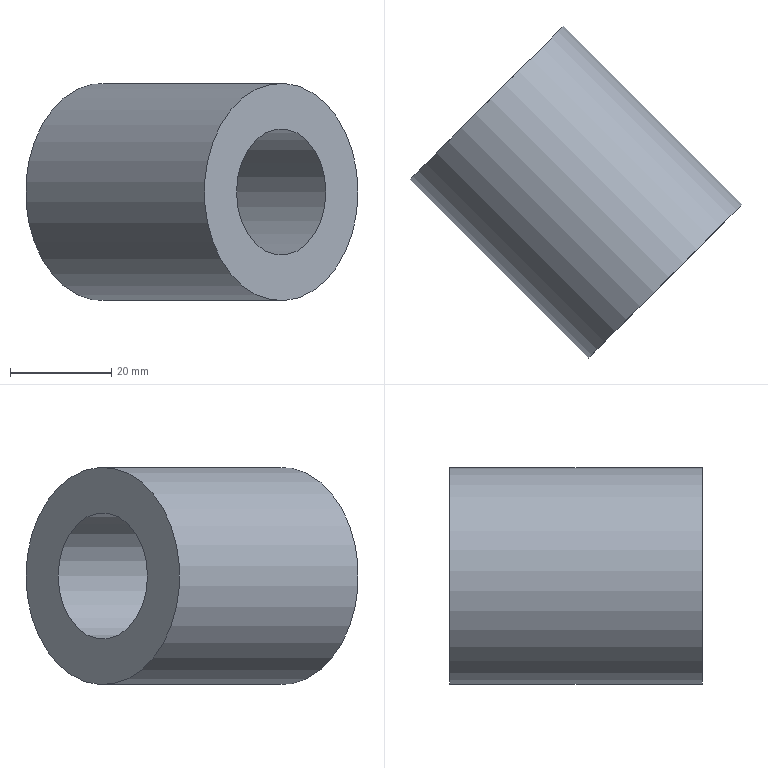Component | NX | INCL_SUPP_FRAME_CONN_COL_2 | 1 solid | 4 faces | box 65.76 x 65.76 x 43 mm | volume 48066 mm3 | cylinder 2 | plane 2 | commonest cylinder face diameters 43 x1 25 x1
STEP:
#1=CARTESIAN_POINT('',(0.,0.,0.));
#2=DIRECTION('',(0.,0.,1.));
#3=DIRECTION('',(1.,0.,0.));
#4=AXIS2_PLACEMENT_3D('',#1,#2,#3);
#5=CARTESIAN_POINT('',(-786.016,863.173,-601.5));
#6=VERTEX_POINT('',#5);
#7=CARTESIAN_POINT('',(-801.219,847.97,-601.5));
#8=DIRECTION('',(0.7071,-0.7071,0.));
#9=DIRECTION('',(0.7071,0.7071,0.));
#10=AXIS2_PLACEMENT_3D('',#7,#8,#9);
#11=CIRCLE('',#10,21.5);
#12=CARTESIAN_POINT('',(-801.219,847.97,-601.5));
#13=DIRECTION('',(0.7071,-0.7071,0.));
#14=DIRECTION('',(-0.7071,-0.7071,0.));
#15=AXIS2_PLACEMENT_3D('',#12,#13,#14);
#16=CYLINDRICAL_SURFACE('',#15,21.5);
#17=CARTESIAN_POINT('',(3.142,0.));
#18=DIRECTION('',(1.,0.));
#19=VECTOR('',#18,1.);
#20=LINE('',#17,#19);
#21=(GEOMETRIC_REPRESENTATION_CONTEXT(2)PARAMETRIC_REPRESENTATION_CONTEXT()REPRESENTATION_CONTEXT('',''));
#22=DEFINITIONAL_REPRESENTATION('',(#20),#21);
#23=PCURVE('',#16,#22);
#24=CARTESIAN_POINT('',(-801.219,847.97,-601.5));
#25=DIRECTION('',(0.7071,-0.7071,0.));
#26=DIRECTION('',(-0.7071,-0.7071,0.));
#27=AXIS2_PLACEMENT_3D('',#24,#25,#26);
#28=PLANE('',#27);
#29=CARTESIAN_POINT('',(0.,0.));
#30=DIRECTION('',(-1.,0.));
#31=AXIS2_PLACEMENT_2D('',#29,#30);
#32=CIRCLE('',#31,21.5);
#33=(GEOMETRIC_REPRESENTATION_CONTEXT(2)PARAMETRIC_REPRESENTATION_CONTEXT()REPRESENTATION_CONTEXT('',''));
#34=DEFINITIONAL_REPRESENTATION('',(#32),#33);
#35=PCURVE('',#28,#34);
#36=SURFACE_CURVE('',#11,(#23,#35),.PCURVE_S1.);
#37=EDGE_CURVE('',#6,#6,#36,.T.);
#38=ORIENTED_EDGE('',*,*,#37,.T.);
#39=CARTESIAN_POINT('',(-750.661,827.817,-601.5));
#40=VERTEX_POINT('',#39);
#41=CARTESIAN_POINT('',(-786.016,863.173,-601.5));
#42=CARTESIAN_POINT('',(-750.661,827.817,-601.5));
#43=B_SPLINE_CURVE_WITH_KNOTS('',1,(#41,#42),.UNSPECIFIED.,.F.,.F.,(2,2),(0.,50.),.PIECEWISE_BEZIER_KNOTS.);
#44=CARTESIAN_POINT('',(9.425,0.));
#45=DIRECTION('',(0.,1.));
#46=VECTOR('',#45,1.);
#47=LINE('',#44,#46);
#48=(GEOMETRIC_REPRESENTATION_CONTEXT(2)PARAMETRIC_REPRESENTATION_CONTEXT()REPRESENTATION_CONTEXT('',''));
#49=DEFINITIONAL_REPRESENTATION('',(#47),#48);
#50=PCURVE('',#16,#49);
#51=CARTESIAN_POINT('',(3.142,0.));
#52=DIRECTION('',(0.,1.));
#53=VECTOR('',#52,1.);
#54=LINE('',#51,#53);
#55=(GEOMETRIC_REPRESENTATION_CONTEXT(2)PARAMETRIC_REPRESENTATION_CONTEXT()REPRESENTATION_CONTEXT('',''));
#56=DEFINITIONAL_REPRESENTATION('',(#54),#55);
#57=PCURVE('',#16,#56);
#58=SEAM_CURVE('',#43,(#50,#57),.PCURVE_S1.);
#59=EDGE_CURVE('',#6,#40,#58,.T.);
#60=ORIENTED_EDGE('',*,*,#59,.T.);
#61=CARTESIAN_POINT('',(-765.864,812.615,-601.5));
#62=DIRECTION('',(0.7071,-0.7071,0.));
#63=DIRECTION('',(0.7071,0.7071,0.));
#64=AXIS2_PLACEMENT_3D('',#61,#62,#63);
#65=CIRCLE('',#64,21.5);
#66=CARTESIAN_POINT('',(3.142,50.));
#67=DIRECTION('',(1.,0.));
#68=VECTOR('',#67,1.);
#69=LINE('',#66,#68);
#70=(GEOMETRIC_REPRESENTATION_CONTEXT(2)PARAMETRIC_REPRESENTATION_CONTEXT()REPRESENTATION_CONTEXT('',''));
#71=DEFINITIONAL_REPRESENTATION('',(#69),#70);
#72=PCURVE('',#16,#71);
#73=CARTESIAN_POINT('',(-765.864,812.615,-601.5));
#74=DIRECTION('',(0.7071,-0.7071,0.));
#75=DIRECTION('',(-0.7071,-0.7071,0.));
#76=AXIS2_PLACEMENT_3D('',#73,#74,#75);
#77=PLANE('',#76);
#78=CARTESIAN_POINT('',(0.,0.));
#79=DIRECTION('',(-1.,0.));
#80=AXIS2_PLACEMENT_2D('',#78,#79);
#81=CIRCLE('',#80,21.5);
#82=(GEOMETRIC_REPRESENTATION_CONTEXT(2)PARAMETRIC_REPRESENTATION_CONTEXT()REPRESENTATION_CONTEXT('',''));
#83=DEFINITIONAL_REPRESENTATION('',(#81),#82);
#84=PCURVE('',#77,#83);
#85=SURFACE_CURVE('',#65,(#72,#84),.PCURVE_S1.);
#86=EDGE_CURVE('',#40,#40,#85,.T.);
#87=ORIENTED_EDGE('',*,*,#86,.F.);
#88=ORIENTED_EDGE('',*,*,#59,.F.);
#89=EDGE_LOOP('',(#38,#60,#87,#88));
#90=FACE_BOUND('',#89,.T.);
#91=ADVANCED_FACE('',(#90),#16,.T.);
#92=CARTESIAN_POINT('',(-792.38,856.809,-601.5));
#93=VERTEX_POINT('',#92);
#94=CARTESIAN_POINT('',(-801.219,847.97,-601.5));
#95=DIRECTION('',(0.7071,-0.7071,0.));
#96=DIRECTION('',(0.7071,0.7071,0.));
#97=AXIS2_PLACEMENT_3D('',#94,#95,#96);
#98=CIRCLE('',#97,12.5);
#99=CARTESIAN_POINT('',(-801.219,847.97,-601.5));
#100=DIRECTION('',(0.7071,-0.7071,0.));
#101=DIRECTION('',(-0.7071,-0.7071,0.));
#102=AXIS2_PLACEMENT_3D('',#99,#100,#101);
#103=CYLINDRICAL_SURFACE('',#102,12.5);
#104=CARTESIAN_POINT('',(3.142,0.));
#105=DIRECTION('',(1.,0.));
#106=VECTOR('',#105,1.);
#107=LINE('',#104,#106);
#108=(GEOMETRIC_REPRESENTATION_CONTEXT(2)PARAMETRIC_REPRESENTATION_CONTEXT()REPRESENTATION_CONTEXT('',''));
#109=DEFINITIONAL_REPRESENTATION('',(#107),#108);
#110=PCURVE('',#103,#109);
#111=CARTESIAN_POINT('',(0.,0.));
#112=DIRECTION('',(-1.,0.));
#113=AXIS2_PLACEMENT_2D('',#111,#112);
#114=CIRCLE('',#113,12.5);
#115=(GEOMETRIC_REPRESENTATION_CONTEXT(2)PARAMETRIC_REPRESENTATION_CONTEXT()REPRESENTATION_CONTEXT('',''));
#116=DEFINITIONAL_REPRESENTATION('',(#114),#115);
#117=PCURVE('',#28,#116);
#118=SURFACE_CURVE('',#98,(#110,#117),.PCURVE_S1.);
#119=EDGE_CURVE('',#93,#93,#118,.T.);
#120=ORIENTED_EDGE('',*,*,#119,.T.);
#121=CARTESIAN_POINT('',(-757.025,821.453,-601.5));
#122=VERTEX_POINT('',#121);
#123=CARTESIAN_POINT('',(-792.38,856.809,-601.5));
#124=CARTESIAN_POINT('',(-757.025,821.453,-601.5));
#125=B_SPLINE_CURVE_WITH_KNOTS('',1,(#123,#124),.UNSPECIFIED.,.F.,.F.,(2,2),(0.,50.),.PIECEWISE_BEZIER_KNOTS.);
#126=CARTESIAN_POINT('',(9.425,0.));
#127=DIRECTION('',(0.,1.));
#128=VECTOR('',#127,1.);
#129=LINE('',#126,#128);
#130=(GEOMETRIC_REPRESENTATION_CONTEXT(2)PARAMETRIC_REPRESENTATION_CONTEXT()REPRESENTATION_CONTEXT('',''));
#131=DEFINITIONAL_REPRESENTATION('',(#129),#130);
#132=PCURVE('',#103,#131);
#133=CARTESIAN_POINT('',(3.142,0.));
#134=DIRECTION('',(0.,1.));
#135=VECTOR('',#134,1.);
#136=LINE('',#133,#135);
#137=(GEOMETRIC_REPRESENTATION_CONTEXT(2)PARAMETRIC_REPRESENTATION_CONTEXT()REPRESENTATION_CONTEXT('',''));
#138=DEFINITIONAL_REPRESENTATION('',(#136),#137);
#139=PCURVE('',#103,#138);
#140=SEAM_CURVE('',#125,(#132,#139),.PCURVE_S1.);
#141=EDGE_CURVE('',#93,#122,#140,.T.);
#142=ORIENTED_EDGE('',*,*,#141,.T.);
#143=CARTESIAN_POINT('',(-765.864,812.615,-601.5));
#144=DIRECTION('',(0.7071,-0.7071,0.));
#145=DIRECTION('',(0.7071,0.7071,0.));
#146=AXIS2_PLACEMENT_3D('',#143,#144,#145);
#147=CIRCLE('',#146,12.5);
#148=CARTESIAN_POINT('',(3.142,50.));
#149=DIRECTION('',(1.,0.));
#150=VECTOR('',#149,1.);
#151=LINE('',#148,#150);
#152=(GEOMETRIC_REPRESENTATION_CONTEXT(2)PARAMETRIC_REPRESENTATION_CONTEXT()REPRESENTATION_CONTEXT('',''));
#153=DEFINITIONAL_REPRESENTATION('',(#151),#152);
#154=PCURVE('',#103,#153);
#155=CARTESIAN_POINT('',(0.,0.));
#156=DIRECTION('',(-1.,0.));
#157=AXIS2_PLACEMENT_2D('',#155,#156);
#158=CIRCLE('',#157,12.5);
#159=(GEOMETRIC_REPRESENTATION_CONTEXT(2)PARAMETRIC_REPRESENTATION_CONTEXT()REPRESENTATION_CONTEXT('',''));
#160=DEFINITIONAL_REPRESENTATION('',(#158),#159);
#161=PCURVE('',#77,#160);
#162=SURFACE_CURVE('',#147,(#154,#161),.PCURVE_S1.);
#163=EDGE_CURVE('',#122,#122,#162,.T.);
#164=ORIENTED_EDGE('',*,*,#163,.F.);
#165=ORIENTED_EDGE('',*,*,#141,.F.);
#166=EDGE_LOOP('',(#120,#142,#164,#165));
#167=FACE_BOUND('',#166,.F.);
#168=ADVANCED_FACE('',(#167),#103,.F.);
#169=ORIENTED_EDGE('',*,*,#37,.F.);
#170=EDGE_LOOP('',(#169));
#171=FACE_BOUND('',#170,.T.);
#172=ORIENTED_EDGE('',*,*,#119,.T.);
#173=EDGE_LOOP('',(#172));
#174=FACE_BOUND('',#173,.T.);
#175=ADVANCED_FACE('',(#171,#174),#28,.F.);
#176=ORIENTED_EDGE('',*,*,#86,.T.);
#177=EDGE_LOOP('',(#176));
#178=FACE_BOUND('',#177,.T.);
#179=ORIENTED_EDGE('',*,*,#163,.F.);
#180=EDGE_LOOP('',(#179));
#181=FACE_BOUND('',#180,.T.);
#182=ADVANCED_FACE('',(#178,#181),#77,.T.);
#183=CLOSED_SHELL('',(#91,#168,#175,#182));
#184=MANIFOLD_SOLID_BREP('',#183);
#185=(LENGTH_UNIT()NAMED_UNIT(*)SI_UNIT(.MILLI.,.METRE.));
#186=UNCERTAINTY_MEASURE_WITH_UNIT(LENGTH_MEASURE(0.00001),#185,'','');
#187=(NAMED_UNIT(*)PLANE_ANGLE_UNIT()SI_UNIT($,.RADIAN.));
#188=(NAMED_UNIT(*)SI_UNIT($,.STERADIAN.)SOLID_ANGLE_UNIT());
#189=(GEOMETRIC_REPRESENTATION_CONTEXT(3)GLOBAL_UNCERTAINTY_ASSIGNED_CONTEXT((#186))GLOBAL_UNIT_ASSIGNED_CONTEXT((#185,#187,#188))REPRESENTATION_CONTEXT('',''));
#190=ADVANCED_BREP_SHAPE_REPRESENTATION('',(#4,#184),#189);